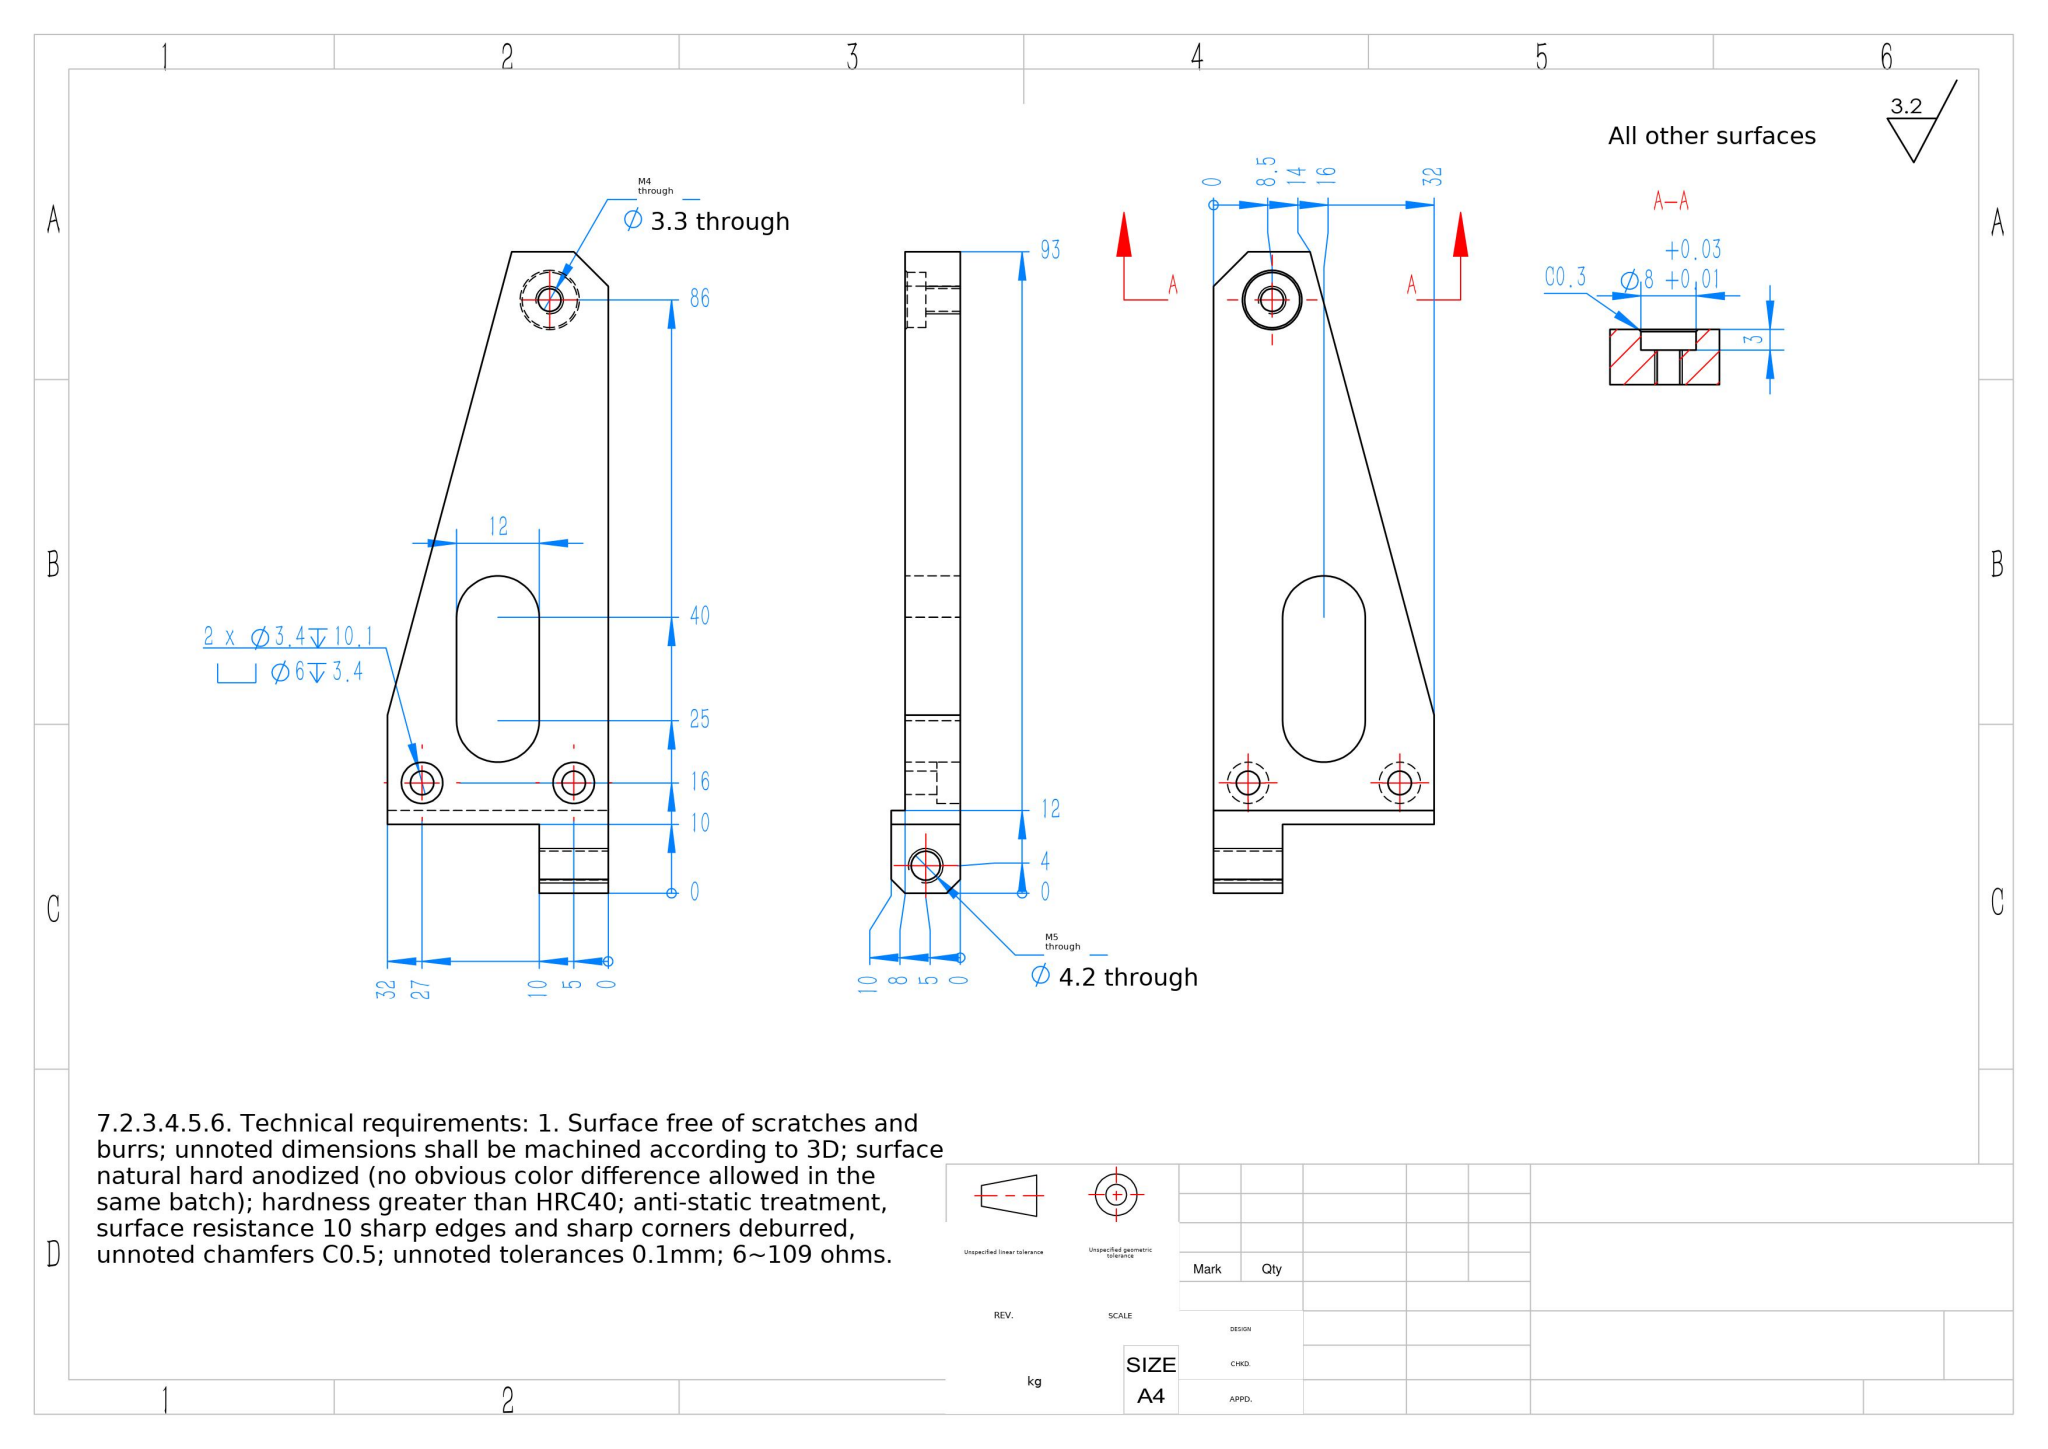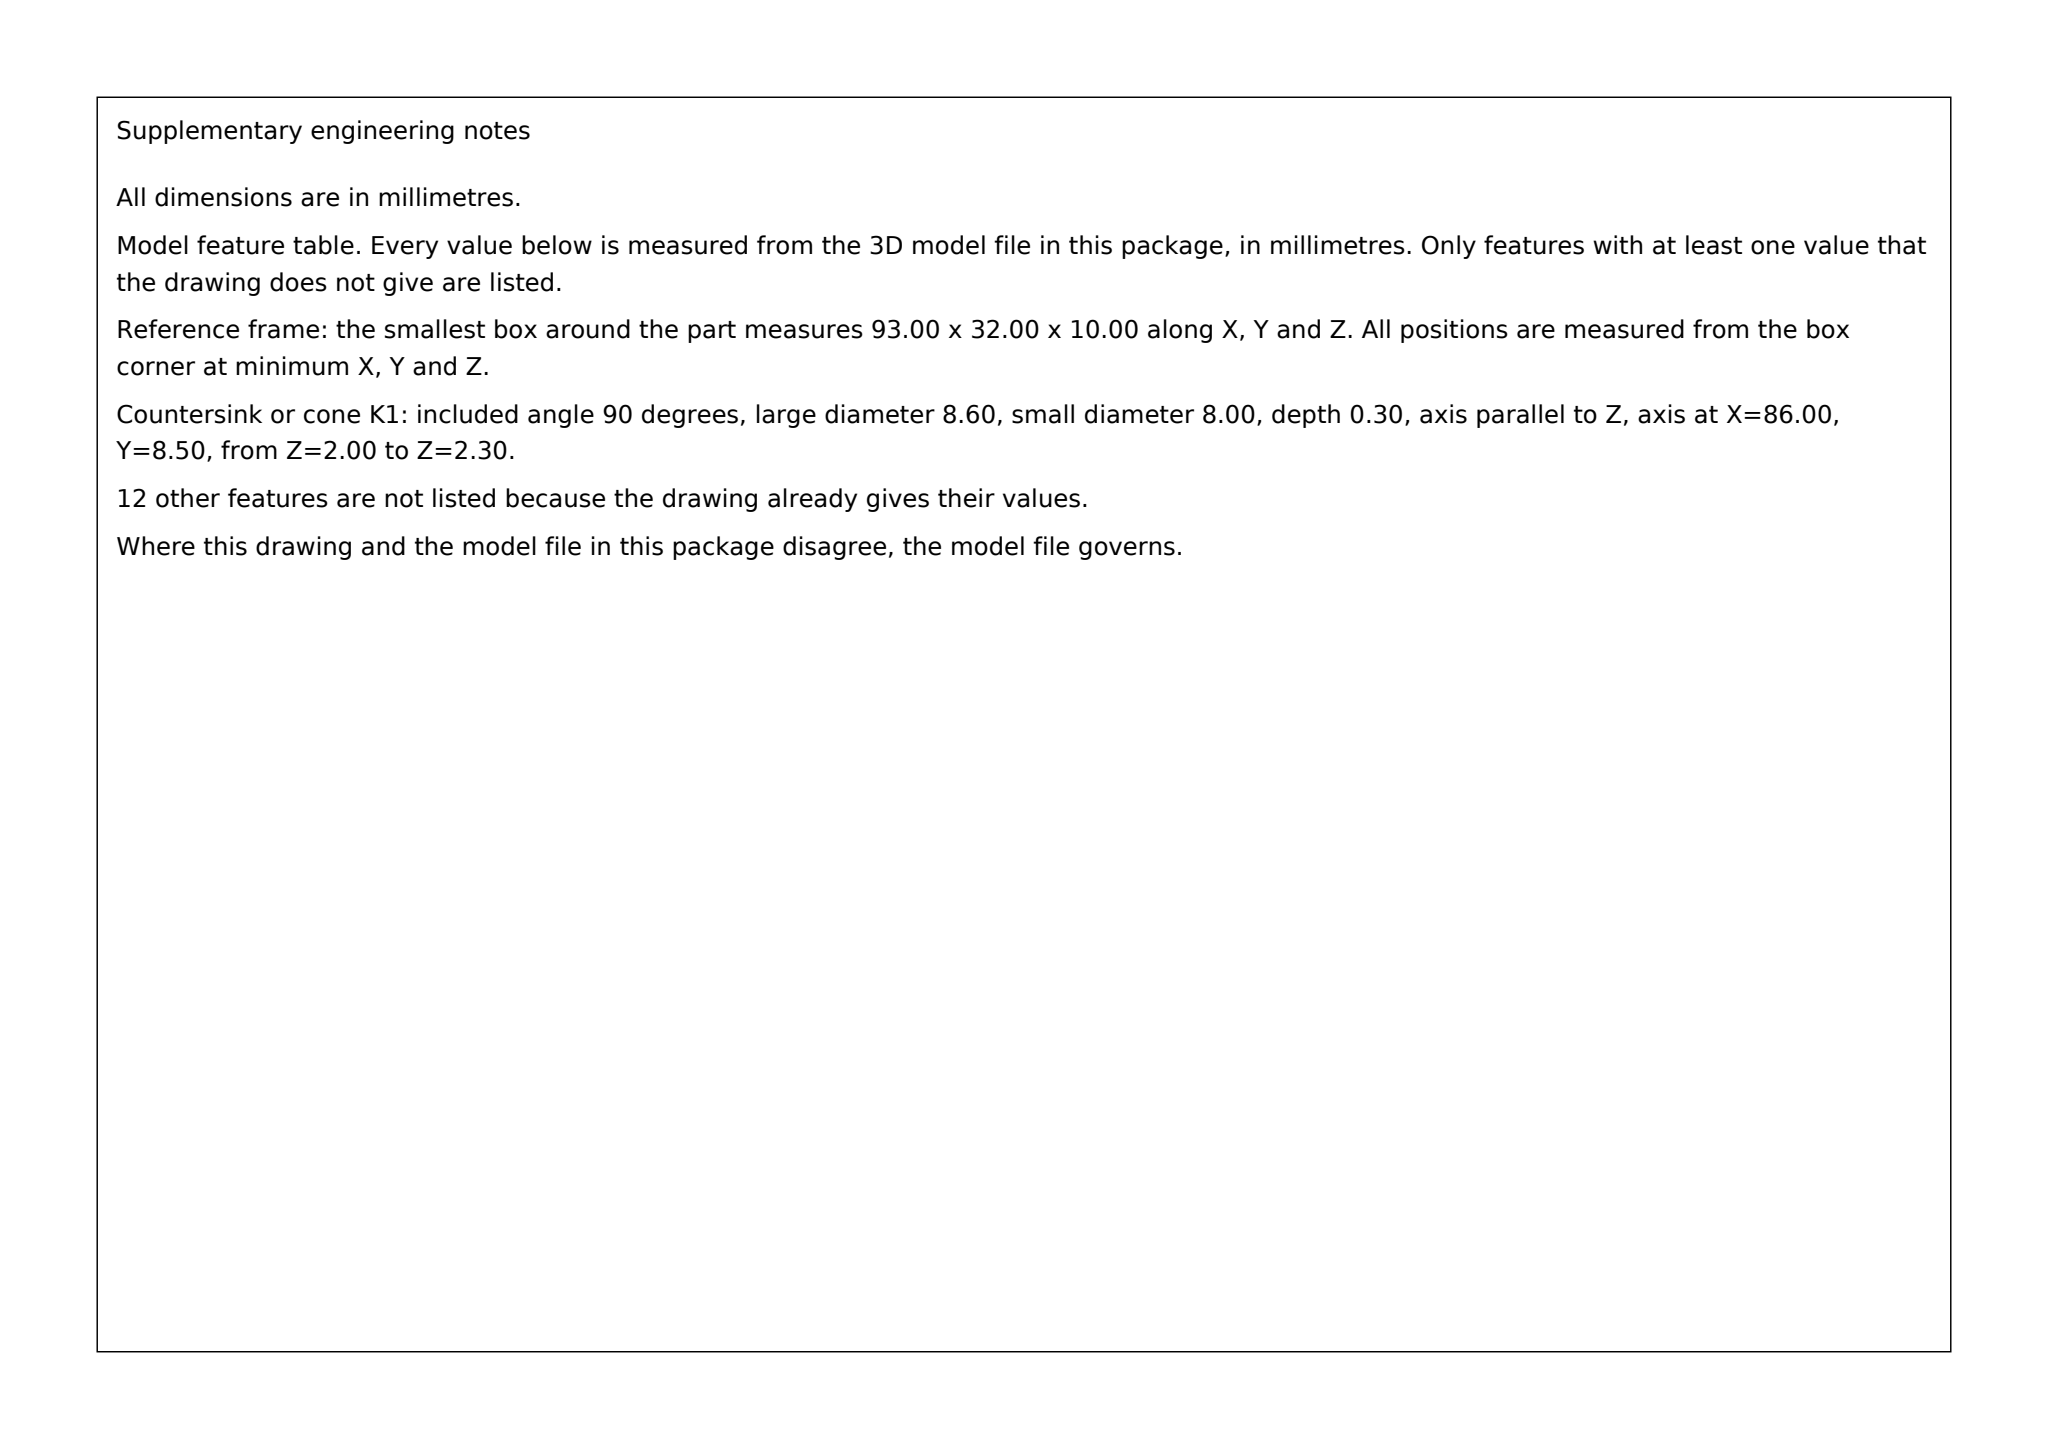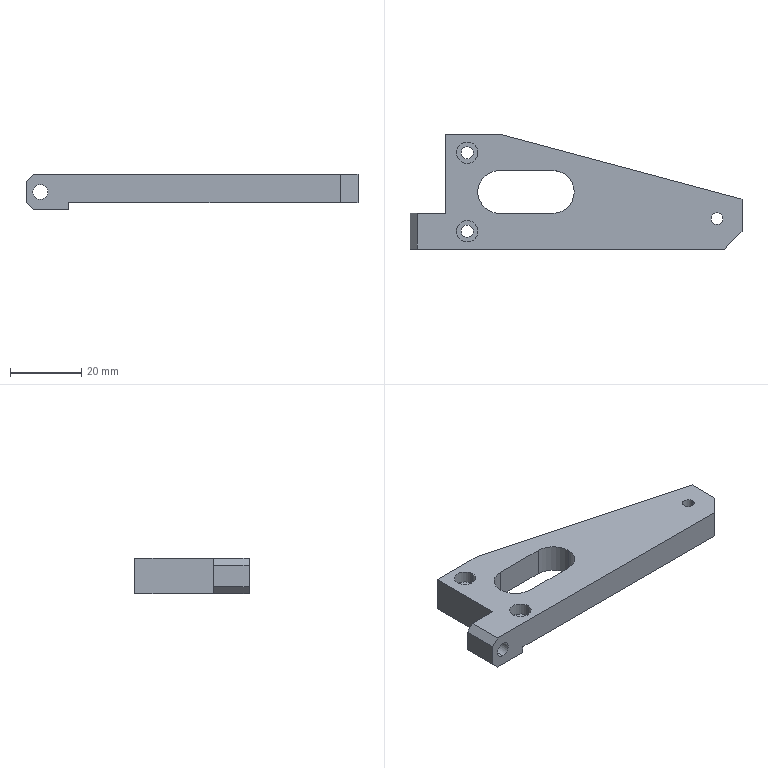Part | SolidWorks | mm | 1 solid | 38 faces | box 93 x 32 x 10 mm | volume 14445 mm3 | plane 19 | cylinder 17 | cone 2 | commonest cylinder face diameters 6 x4 3.4 x4 12 x3 4.2 x2 8 x2 3.3 x2
build123d program:
from build123d import *

# Parameters (mm, degrees)
SKETCH1_W                                         = 83
SKETCH1_H                                         = 32
BOSS_EXTRUDE1_DEPTH                               = 5
SKETCH2_W                                         = 100
SKETCH2_H                                         = 2
CUT_EXTRUDE4_DEPTH                                = 53.643
CHAMFER1_SIZE                                     = 5
M4_TAPPED_HOLE1_D                                 = 3.3
SKETCH8_R                                         = 4
CUT_EXTRUDE5_DEPTH                                = 3
HOLE_SIZE_ACCORDING_TO_HEXAGON_SOCKET_D           = 3.4
HOLE_SIZE_ACCORDING_TO_HEXAGON_SOCKET_DEPTH       = 10.1
HOLE_SIZE_ACCORDING_TO_HEXAGON_SOCKET_CBORE_D     = 6
HOLE_SIZE_ACCORDING_TO_HEXAGON_SOCKET_CBORE_DEPTH = 3.4
HOLE_SIZE_ACCORDING_TO_HEXAGON_SOCKET_TIP         = 1.021
CUT_EXTRUDE6_DEPTH                                = 46.588
SKETCH12_W                                        = 10
SKETCH12_H                                        = 10
BOSS_EXTRUDE2_DEPTH                               = 10
CHAMFER3_SIZE                                     = 2
M5_TAPPED_HOLE1_D                                 = 4.2
CHAMFER4_SIZE                                     = 18
CHAMFER4_SIZE2                                    = 67.177
CHAMFER5_SIZE                                     = 0.3


with BuildPart() as part:
    # Sketch1 → Boss-Extrude1 (new, symmetric)
    with BuildSketch(Plane.XY):
        Rectangle(SKETCH1_W, SKETCH1_H)
    extrude(amount=BOSS_EXTRUDE1_DEPTH, both=True)

    # Sketch2 → Cut-Extrude4 (cut, through all)
    with BuildSketch(Plane.XZ.offset(16)):
        with Locations((10.5, -4)):
            Rectangle(SKETCH2_W, SKETCH2_H)
    extrude(amount=-CUT_EXTRUDE4_DEPTH, mode=Mode.SUBTRACT)

    # Chamfer1
    chamfer1_edges = [part.edges().sort_by_distance(p)[0] for p in [
        (41.5, -16, 1),
    ]]
    chamfer(chamfer1_edges, length=CHAMFER1_SIZE)

    # M4 Tapped Hole1 (through all)
    with Locations(Plane(origin=(0, 0, -5), x_dir=(-1, 0, 0), z_dir=(0, 0, -1))):
        with Locations((-34.5, -7.5)):
            Hole(M4_TAPPED_HOLE1_D / 2)

    # Sketch8 → Cut-Extrude5 (cut)
    with BuildSketch(Plane(origin=(0, 0, -3), x_dir=(-1, 0, 0), z_dir=(0, 0, -1))):
        with Locations((-34.5, -7.5)):
            Circle(SKETCH8_R)
    extrude(amount=-CUT_EXTRUDE5_DEPTH, mode=Mode.SUBTRACT)

    # Hole Size _ according to_ Hexagon Socket
    with Locations(Plane.XY.offset(5)):
        with Locations((-35.5, 11), (-35.5, -11)):
            CounterBoreHole(HOLE_SIZE_ACCORDING_TO_HEXAGON_SOCKET_D / 2, HOLE_SIZE_ACCORDING_TO_HEXAGON_SOCKET_CBORE_D / 2, HOLE_SIZE_ACCORDING_TO_HEXAGON_SOCKET_CBORE_DEPTH, depth=HOLE_SIZE_ACCORDING_TO_HEXAGON_SOCKET_DEPTH)
            with Locations((0, 0, -(HOLE_SIZE_ACCORDING_TO_HEXAGON_SOCKET_DEPTH + HOLE_SIZE_ACCORDING_TO_HEXAGON_SOCKET_TIP / 2))):  # 118° drill point
                Cone(0, HOLE_SIZE_ACCORDING_TO_HEXAGON_SOCKET_D / 2, HOLE_SIZE_ACCORDING_TO_HEXAGON_SOCKET_TIP, mode=Mode.SUBTRACT)

    # Sketch11 → Cut-Extrude6 (cut, through all)
    with BuildSketch(Plane.XY.offset(5)):
        with BuildLine():
            Line((-11.5, -6), (-26.5, -6))
            ThreePointArc((-26.5, -6), (-32.5, 0), (-26.5, 6))
            Line((-26.5, 6), (-11.5, 6))
            ThreePointArc((-11.5, 6), (-5.5, 0), (-11.5, -6))
        make_face()
    extrude(amount=-CUT_EXTRUDE6_DEPTH, mode=Mode.SUBTRACT)

    # Sketch12 → Boss-Extrude2 (add)
    with BuildSketch(Plane.ZY.offset(41.5)):
        with Locations((0, -11)):
            Rectangle(SKETCH12_W, SKETCH12_H)
    extrude(amount=BOSS_EXTRUDE2_DEPTH)

    # Chamfer3
    chamfer3_edges = [part.edges().sort_by_distance(p)[0] for p in [
        (-51.5, -11, 5),
        (-51.5, -11, -5),
    ]]
    chamfer(chamfer3_edges, length=CHAMFER3_SIZE)

    # M5 Tapped Hole1 (through all)
    with Locations(Plane(origin=(0, -16, 0), x_dir=(-1, 0, 0), z_dir=(0, -1, 0))):
        with Locations((47.5, 0)):
            Hole(M5_TAPPED_HOLE1_D / 2)

    # Chamfer4
    chamfer4_edges = [part.edges().sort_by_distance(p)[0] for p in [
        (41.5, 16, 1),
    ]]
    chamfer4_side = [part.faces().sort_by_distance(p)[0] for p in [
        (41.5, 2.5, 1),
    ]]
    chamfer(chamfer4_edges, length=CHAMFER4_SIZE, length2=CHAMFER4_SIZE2, reference=chamfer4_side[0])

    # Chamfer5
    chamfer5_edges = [part.edges().sort_by_distance(p)[0] for p in [
        (38.5, -7.5, -3),
    ]]
    chamfer(chamfer5_edges, length=CHAMFER5_SIZE)


solid = part.part